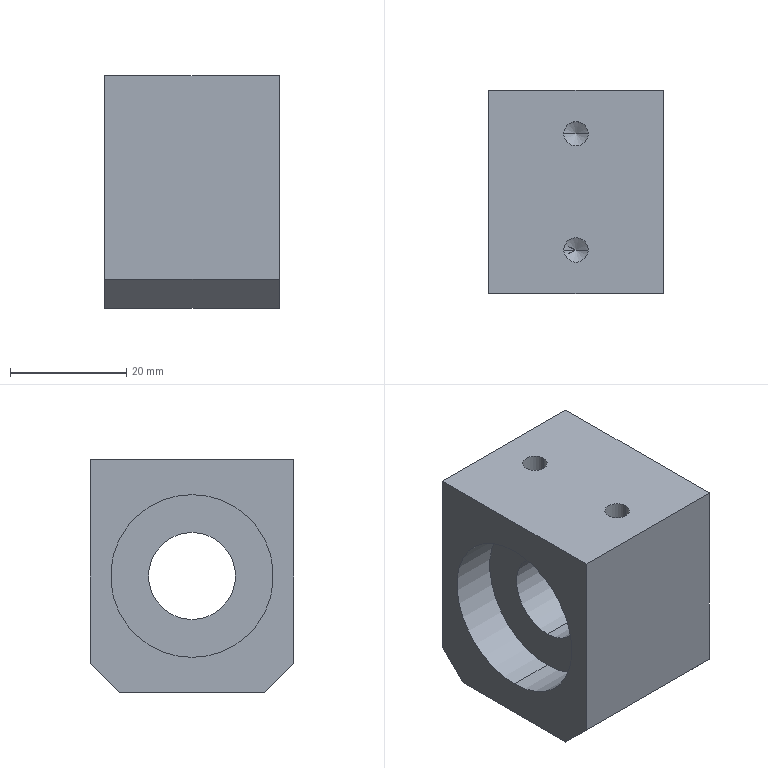Component | SolidWorks | ElectricalBoxAssembly2-1_AngleSensorComponentAssembly3-1_BearingHousing2-1 | 1 solid | 24 faces | box 30 x 35 x 40 mm | volume 28569 mm3 | cylinder 10 | plane 10 | cone 4 | commonest cylinder face diameters 4.2 x4 28 x4 15 x2
build123d program:
from build123d import *

# Parameters (mm, degrees)
SKETCH1_W             = 40
SKETCH1_H             = 35
BOSS_EXTRUDE1_DEPTH   = 15
SKETCH2_R             = 14
CUT_EXTRUDE1_DEPTH    = 8
SKETCH3_R             = 7.5
CUT_EXTRUDE2_DEPTH    = 35.5
M5_TAPPED_HOLE1_D     = 4.2
M5_TAPPED_HOLE1_DEPTH = 12.4
M5_TAPPED_HOLE1_TIP   = 1.262
CHAMFER1_SIZE         = 5


with BuildPart() as part:
    # Sketch1 → Boss-Extrude1 (new, symmetric)
    with BuildSketch(Plane.XY):
        Rectangle(SKETCH1_W, SKETCH1_H)
    extrude(amount=BOSS_EXTRUDE1_DEPTH, both=True)

    # Sketch2 → Cut-Extrude1 (cut)
    with BuildSketch(Plane.XY.offset(15)):
        Circle(SKETCH2_R)
    cut_extrude1 = extrude(amount=-CUT_EXTRUDE1_DEPTH, mode=Mode.SUBTRACT)

    # Mirror1: Cut-Extrude1 across plane
    add(cut_extrude1.mirror(Plane.XY), mode=Mode.SUBTRACT)

    # Sketch3 → Cut-Extrude2 (cut, through all)
    with BuildSketch(Plane.XY.offset(7)):
        Circle(SKETCH3_R)
    extrude(amount=-CUT_EXTRUDE2_DEPTH, mode=Mode.SUBTRACT)

    # M5 Tapped Hole1
    with Locations(Plane(origin=(20, 0, 0), x_dir=(0, 0, -1), z_dir=(1, 0, 0))):
        with Locations((0, 10), (0, -10)):
            Hole(M5_TAPPED_HOLE1_D / 2, depth=M5_TAPPED_HOLE1_DEPTH)
            with Locations((0, 0, -(M5_TAPPED_HOLE1_DEPTH + M5_TAPPED_HOLE1_TIP / 2))):  # 118° drill point
                Cone(0, M5_TAPPED_HOLE1_D / 2, M5_TAPPED_HOLE1_TIP, mode=Mode.SUBTRACT)

    # Chamfer1
    chamfer1_edges = [part.edges().sort_by_distance(p)[0] for p in [
        (-20, -17.5, 0),
        (-20, 17.5, 0),
    ]]
    chamfer(chamfer1_edges, length=CHAMFER1_SIZE)


solid = part.part

# Placed as in the assembly
solid = solid.moved(Location((824.115, 214.666, 1746.399), (0, -90, 0)))
STEP:
#1=COLOUR_RGB('',0.7922,0.8196,0.9333);
#2=FILL_AREA_STYLE_COLOUR('',#1);
#3=FILL_AREA_STYLE('',(#2));
#4=SURFACE_STYLE_FILL_AREA(#3);
#5=SURFACE_SIDE_STYLE('',(#4));
#6=SURFACE_STYLE_USAGE(.BOTH.,#5);
#7=PRESENTATION_STYLE_ASSIGNMENT((#6));
#8=CARTESIAN_POINT('',(32.363,8.845,69.055));
#9=VERTEX_POINT('',#8);
#10=CARTESIAN_POINT('',(32.528,8.845,69.055));
#11=VERTEX_POINT('',#10);
#12=CARTESIAN_POINT('',(32.445,8.845,69.055));
#13=DIRECTION('',(0.,0.,1.));
#14=DIRECTION('',(1.,0.,0.));
#15=AXIS2_PLACEMENT_3D('',#12,#13,#14);
#16=CIRCLE('',#15,0.08268);
#17=EDGE_CURVE('',#9,#11,#16,.T.);
#18=ORIENTED_EDGE('',*,*,#17,.F.);
#19=CARTESIAN_POINT('',(32.363,8.845,69.543));
#20=VERTEX_POINT('',#19);
#21=CARTESIAN_POINT('',(32.363,8.845,69.543));
#22=DIRECTION('',(0.,0.,1.));
#23=VECTOR('',#22,39.37);
#24=LINE('',#21,#23);
#25=EDGE_CURVE('',#9,#20,#24,.T.);
#26=ORIENTED_EDGE('',*,*,#25,.T.);
#27=CARTESIAN_POINT('',(32.528,8.845,69.543));
#28=VERTEX_POINT('',#27);
#29=CARTESIAN_POINT('',(32.445,8.845,69.543));
#30=DIRECTION('',(0.,0.,1.));
#31=DIRECTION('',(1.,0.,0.));
#32=AXIS2_PLACEMENT_3D('',#29,#30,#31);
#33=CIRCLE('',#32,0.08268);
#34=EDGE_CURVE('',#20,#28,#33,.T.);
#35=ORIENTED_EDGE('',*,*,#34,.T.);
#36=CARTESIAN_POINT('',(32.528,8.845,69.543));
#37=DIRECTION('',(0.,0.,1.));
#38=VECTOR('',#37,39.37);
#39=LINE('',#36,#38);
#40=EDGE_CURVE('',#11,#28,#39,.T.);
#41=ORIENTED_EDGE('',*,*,#40,.F.);
#42=EDGE_LOOP('',(#18,#26,#35,#41));
#43=FACE_OUTER_BOUND('',#42,.T.);
#44=CARTESIAN_POINT('',(32.445,8.845,69.543));
#45=DIRECTION('',(0.,0.,1.));
#46=DIRECTION('',(1.,0.,0.));
#47=AXIS2_PLACEMENT_3D('',#44,#45,#46);
#48=CYLINDRICAL_SURFACE('',#47,0.08268);
#49=ADVANCED_FACE('',(#43),#48,.F.);
#50=CARTESIAN_POINT('',(32.445,8.845,69.005));
#51=VERTEX_POINT('',#50);
#52=CARTESIAN_POINT('',(32.528,8.845,69.055));
#53=DIRECTION('',(0.8572,0.,0.515));
#54=VECTOR('',#53,39.37);
#55=LINE('',#52,#54);
#56=EDGE_CURVE('',#51,#11,#55,.T.);
#57=ORIENTED_EDGE('',*,*,#56,.F.);
#58=CARTESIAN_POINT('',(32.363,8.845,69.055));
#59=DIRECTION('',(-0.8572,0.,0.515));
#60=VECTOR('',#59,39.37);
#61=LINE('',#58,#60);
#62=EDGE_CURVE('',#51,#9,#61,.T.);
#63=ORIENTED_EDGE('',*,*,#62,.T.);
#64=ORIENTED_EDGE('',*,*,#17,.T.);
#65=EDGE_LOOP('',(#57,#63,#64));
#66=FACE_OUTER_BOUND('',#65,.T.);
#67=CARTESIAN_POINT('',(32.445,8.845,69.055));
#68=DIRECTION('',(0.,0.,1.));
#69=DIRECTION('',(1.,0.,0.));
#70=AXIS2_PLACEMENT_3D('',#67,#68,#69);
#71=CONICAL_SURFACE('',#70,0.08268,1.03);
#72=ADVANCED_FACE('',(#66),#71,.F.);
#73=CARTESIAN_POINT('',(32.363,8.058,69.055));
#74=VERTEX_POINT('',#73);
#75=CARTESIAN_POINT('',(32.528,8.058,69.055));
#76=VERTEX_POINT('',#75);
#77=CARTESIAN_POINT('',(32.445,8.058,69.055));
#78=DIRECTION('',(0.,0.,1.));
#79=DIRECTION('',(1.,0.,0.));
#80=AXIS2_PLACEMENT_3D('',#77,#78,#79);
#81=CIRCLE('',#80,0.08268);
#82=EDGE_CURVE('',#74,#76,#81,.T.);
#83=ORIENTED_EDGE('',*,*,#82,.F.);
#84=CARTESIAN_POINT('',(32.363,8.058,69.543));
#85=VERTEX_POINT('',#84);
#86=CARTESIAN_POINT('',(32.363,8.058,69.543));
#87=DIRECTION('',(0.,0.,1.));
#88=VECTOR('',#87,39.37);
#89=LINE('',#86,#88);
#90=EDGE_CURVE('',#74,#85,#89,.T.);
#91=ORIENTED_EDGE('',*,*,#90,.T.);
#92=CARTESIAN_POINT('',(32.528,8.058,69.543));
#93=VERTEX_POINT('',#92);
#94=CARTESIAN_POINT('',(32.445,8.058,69.543));
#95=DIRECTION('',(0.,0.,1.));
#96=DIRECTION('',(1.,0.,0.));
#97=AXIS2_PLACEMENT_3D('',#94,#95,#96);
#98=CIRCLE('',#97,0.08268);
#99=EDGE_CURVE('',#85,#93,#98,.T.);
#100=ORIENTED_EDGE('',*,*,#99,.T.);
#101=CARTESIAN_POINT('',(32.528,8.058,69.543));
#102=DIRECTION('',(0.,0.,1.));
#103=VECTOR('',#102,39.37);
#104=LINE('',#101,#103);
#105=EDGE_CURVE('',#76,#93,#104,.T.);
#106=ORIENTED_EDGE('',*,*,#105,.F.);
#107=EDGE_LOOP('',(#83,#91,#100,#106));
#108=FACE_OUTER_BOUND('',#107,.T.);
#109=CARTESIAN_POINT('',(32.445,8.058,69.543));
#110=DIRECTION('',(0.,0.,1.));
#111=DIRECTION('',(1.,0.,0.));
#112=AXIS2_PLACEMENT_3D('',#109,#110,#111);
#113=CYLINDRICAL_SURFACE('',#112,0.08268);
#114=ADVANCED_FACE('',(#108),#113,.F.);
#115=CARTESIAN_POINT('',(32.445,8.058,69.005));
#116=VERTEX_POINT('',#115);
#117=CARTESIAN_POINT('',(32.528,8.058,69.055));
#118=DIRECTION('',(0.8572,0.,0.515));
#119=VECTOR('',#118,39.37);
#120=LINE('',#117,#119);
#121=EDGE_CURVE('',#116,#76,#120,.T.);
#122=ORIENTED_EDGE('',*,*,#121,.F.);
#123=CARTESIAN_POINT('',(32.363,8.058,69.055));
#124=DIRECTION('',(-0.8572,0.,0.515));
#125=VECTOR('',#124,39.37);
#126=LINE('',#123,#125);
#127=EDGE_CURVE('',#116,#74,#126,.T.);
#128=ORIENTED_EDGE('',*,*,#127,.T.);
#129=ORIENTED_EDGE('',*,*,#82,.T.);
#130=EDGE_LOOP('',(#122,#128,#129));
#131=FACE_OUTER_BOUND('',#130,.T.);
#132=CARTESIAN_POINT('',(32.445,8.058,69.055));
#133=DIRECTION('',(0.,0.,1.));
#134=DIRECTION('',(1.,0.,0.));
#135=AXIS2_PLACEMENT_3D('',#132,#133,#134);
#136=CONICAL_SURFACE('',#135,0.08268,1.03);
#137=ADVANCED_FACE('',(#131),#136,.F.);
#138=CARTESIAN_POINT('',(32.721,8.451,69.051));
#139=VERTEX_POINT('',#138);
#140=CARTESIAN_POINT('',(32.721,8.451,68.461));
#141=VERTEX_POINT('',#140);
#142=CARTESIAN_POINT('',(32.721,8.451,68.756));
#143=DIRECTION('',(1.,0.,-0.));
#144=DIRECTION('',(-0.,-0.,-1.));
#145=AXIS2_PLACEMENT_3D('',#142,#143,#144);
#146=CIRCLE('',#145,0.2953);
#147=EDGE_CURVE('',#139,#141,#146,.T.);
#148=ORIENTED_EDGE('',*,*,#147,.T.);
#149=CARTESIAN_POINT('',(32.17,8.451,68.461));
#150=VERTEX_POINT('',#149);
#151=CARTESIAN_POINT('',(33.036,8.451,68.461));
#152=DIRECTION('',(-1.,-0.,0.));
#153=VECTOR('',#152,39.37);
#154=LINE('',#151,#153);
#155=EDGE_CURVE('',#141,#150,#154,.T.);
#156=ORIENTED_EDGE('',*,*,#155,.T.);
#157=CARTESIAN_POINT('',(32.17,8.451,69.051));
#158=VERTEX_POINT('',#157);
#159=CARTESIAN_POINT('',(32.17,8.451,68.756));
#160=DIRECTION('',(-1.,-0.,0.));
#161=DIRECTION('',(0.,0.,1.));
#162=AXIS2_PLACEMENT_3D('',#159,#160,#161);
#163=CIRCLE('',#162,0.2953);
#164=EDGE_CURVE('',#150,#158,#163,.T.);
#165=ORIENTED_EDGE('',*,*,#164,.T.);
#166=CARTESIAN_POINT('',(33.036,8.451,69.051));
#167=DIRECTION('',(-1.,-0.,0.));
#168=VECTOR('',#167,39.37);
#169=LINE('',#166,#168);
#170=EDGE_CURVE('',#139,#158,#169,.T.);
#171=ORIENTED_EDGE('',*,*,#170,.F.);
#172=EDGE_LOOP('',(#148,#156,#165,#171));
#173=FACE_OUTER_BOUND('',#172,.T.);
#174=CARTESIAN_POINT('',(33.036,8.451,68.756));
#175=DIRECTION('',(-1.,-0.,0.));
#176=DIRECTION('',(0.,0.,1.));
#177=AXIS2_PLACEMENT_3D('',#174,#175,#176);
#178=CYLINDRICAL_SURFACE('',#177,0.2953);
#179=ADVANCED_FACE('',(#173),#178,.F.);
#180=CARTESIAN_POINT('',(32.721,8.451,68.205));
#181=VERTEX_POINT('',#180);
#182=CARTESIAN_POINT('',(32.721,8.451,69.307));
#183=VERTEX_POINT('',#182);
#184=CARTESIAN_POINT('',(32.721,8.451,68.756));
#185=DIRECTION('',(-1.,-0.,0.));
#186=DIRECTION('',(0.,0.,1.));
#187=AXIS2_PLACEMENT_3D('',#184,#185,#186);
#188=CIRCLE('',#187,0.5512);
#189=EDGE_CURVE('',#181,#183,#188,.T.);
#190=ORIENTED_EDGE('',*,*,#189,.T.);
#191=CARTESIAN_POINT('',(33.036,8.451,69.307));
#192=VERTEX_POINT('',#191);
#193=CARTESIAN_POINT('',(32.721,8.451,69.307));
#194=DIRECTION('',(1.,0.,-0.));
#195=VECTOR('',#194,39.37);
#196=LINE('',#193,#195);
#197=EDGE_CURVE('',#183,#192,#196,.T.);
#198=ORIENTED_EDGE('',*,*,#197,.T.);
#199=CARTESIAN_POINT('',(33.036,8.451,68.205));
#200=VERTEX_POINT('',#199);
#201=CARTESIAN_POINT('',(33.036,8.451,68.756));
#202=DIRECTION('',(-1.,-0.,0.));
#203=DIRECTION('',(0.,0.,1.));
#204=AXIS2_PLACEMENT_3D('',#201,#202,#203);
#205=CIRCLE('',#204,0.5512);
#206=EDGE_CURVE('',#200,#192,#205,.T.);
#207=ORIENTED_EDGE('',*,*,#206,.F.);
#208=CARTESIAN_POINT('',(32.721,8.451,68.205));
#209=DIRECTION('',(1.,0.,-0.));
#210=VECTOR('',#209,39.37);
#211=LINE('',#208,#210);
#212=EDGE_CURVE('',#181,#200,#211,.T.);
#213=ORIENTED_EDGE('',*,*,#212,.F.);
#214=EDGE_LOOP('',(#190,#198,#207,#213));
#215=FACE_OUTER_BOUND('',#214,.T.);
#216=CARTESIAN_POINT('',(32.721,8.451,68.756));
#217=DIRECTION('',(1.,0.,-0.));
#218=DIRECTION('',(-0.,-0.,-1.));
#219=AXIS2_PLACEMENT_3D('',#216,#217,#218);
#220=CYLINDRICAL_SURFACE('',#219,0.5512);
#221=ADVANCED_FACE('',(#215),#220,.F.);
#222=CARTESIAN_POINT('',(32.17,8.451,68.205));
#223=VERTEX_POINT('',#222);
#224=CARTESIAN_POINT('',(32.17,8.451,69.307));
#225=VERTEX_POINT('',#224);
#226=CARTESIAN_POINT('',(32.17,8.451,68.756));
#227=DIRECTION('',(-1.,-0.,0.));
#228=DIRECTION('',(0.,0.,1.));
#229=AXIS2_PLACEMENT_3D('',#226,#227,#228);
#230=CIRCLE('',#229,0.5512);
#231=EDGE_CURVE('',#223,#225,#230,.T.);
#232=ORIENTED_EDGE('',*,*,#231,.F.);
#233=CARTESIAN_POINT('',(31.855,8.451,68.205));
#234=VERTEX_POINT('',#233);
#235=CARTESIAN_POINT('',(32.17,8.451,68.205));
#236=DIRECTION('',(-1.,-0.,0.));
#237=VECTOR('',#236,39.37);
#238=LINE('',#235,#237);
#239=EDGE_CURVE('',#223,#234,#238,.T.);
#240=ORIENTED_EDGE('',*,*,#239,.T.);
#241=CARTESIAN_POINT('',(31.855,8.451,69.307));
#242=VERTEX_POINT('',#241);
#243=CARTESIAN_POINT('',(31.855,8.451,68.756));
#244=DIRECTION('',(-1.,-0.,0.));
#245=DIRECTION('',(0.,0.,1.));
#246=AXIS2_PLACEMENT_3D('',#243,#244,#245);
#247=CIRCLE('',#246,0.5512);
#248=EDGE_CURVE('',#234,#242,#247,.T.);
#249=ORIENTED_EDGE('',*,*,#248,.T.);
#250=CARTESIAN_POINT('',(32.17,8.451,69.307));
#251=DIRECTION('',(-1.,-0.,0.));
#252=VECTOR('',#251,39.37);
#253=LINE('',#250,#252);
#254=EDGE_CURVE('',#225,#242,#253,.T.);
#255=ORIENTED_EDGE('',*,*,#254,.F.);
#256=EDGE_LOOP('',(#232,#240,#249,#255));
#257=FACE_OUTER_BOUND('',#256,.T.);
#258=CARTESIAN_POINT('',(32.17,8.451,68.756));
#259=DIRECTION('',(-1.,-0.,0.));
#260=DIRECTION('',(0.,0.,1.));
#261=AXIS2_PLACEMENT_3D('',#258,#259,#260);
#262=CYLINDRICAL_SURFACE('',#261,0.5512);
#263=ADVANCED_FACE('',(#257),#262,.F.);
#264=CARTESIAN_POINT('',(32.445,8.845,69.543));
#265=DIRECTION('',(0.,0.,1.));
#266=DIRECTION('',(1.,0.,0.));
#267=AXIS2_PLACEMENT_3D('',#264,#265,#266);
#268=CIRCLE('',#267,0.08268);
#269=EDGE_CURVE('',#28,#20,#268,.T.);
#270=ORIENTED_EDGE('',*,*,#269,.F.);
#271=ORIENTED_EDGE('',*,*,#34,.F.);
#272=EDGE_LOOP('',(#270,#271));
#273=FACE_BOUND('',#272,.T.);
#274=CARTESIAN_POINT('',(32.445,8.058,69.543));
#275=DIRECTION('',(0.,0.,1.));
#276=DIRECTION('',(1.,0.,0.));
#277=AXIS2_PLACEMENT_3D('',#274,#275,#276);
#278=CIRCLE('',#277,0.08268);
#279=EDGE_CURVE('',#93,#85,#278,.T.);
#280=ORIENTED_EDGE('',*,*,#279,.F.);
#281=ORIENTED_EDGE('',*,*,#99,.F.);
#282=EDGE_LOOP('',(#280,#281));
#283=FACE_BOUND('',#282,.T.);
#284=CARTESIAN_POINT('',(33.036,7.762,69.543));
#285=VERTEX_POINT('',#284);
#286=CARTESIAN_POINT('',(33.036,9.14,69.543));
#287=VERTEX_POINT('',#286);
#288=CARTESIAN_POINT('',(33.036,9.14,69.543));
#289=DIRECTION('',(-0.,1.,-0.));
#290=VECTOR('',#289,39.37);
#291=LINE('',#288,#290);
#292=EDGE_CURVE('',#285,#287,#291,.T.);
#293=ORIENTED_EDGE('',*,*,#292,.T.);
#294=CARTESIAN_POINT('',(31.855,9.14,69.543));
#295=VERTEX_POINT('',#294);
#296=CARTESIAN_POINT('',(31.855,9.14,69.543));
#297=DIRECTION('',(1.,0.,-0.));
#298=VECTOR('',#297,39.37);
#299=LINE('',#296,#298);
#300=EDGE_CURVE('',#295,#287,#299,.T.);
#301=ORIENTED_EDGE('',*,*,#300,.F.);
#302=CARTESIAN_POINT('',(31.855,7.762,69.543));
#303=VERTEX_POINT('',#302);
#304=CARTESIAN_POINT('',(31.855,9.14,69.543));
#305=DIRECTION('',(-0.,1.,-0.));
#306=VECTOR('',#305,39.37);
#307=LINE('',#304,#306);
#308=EDGE_CURVE('',#303,#295,#307,.T.);
#309=ORIENTED_EDGE('',*,*,#308,.F.);
#310=CARTESIAN_POINT('',(31.855,7.762,69.543));
#311=DIRECTION('',(1.,0.,-0.));
#312=VECTOR('',#311,39.37);
#313=LINE('',#310,#312);
#314=EDGE_CURVE('',#303,#285,#313,.T.);
#315=ORIENTED_EDGE('',*,*,#314,.T.);
#316=EDGE_LOOP('',(#293,#301,#309,#315));
#317=FACE_OUTER_BOUND('',#316,.T.);
#318=CARTESIAN_POINT('',(31.855,9.14,69.543));
#319=DIRECTION('',(-0.,-0.,-1.));
#320=DIRECTION('',(0.,-1.,0.));
#321=AXIS2_PLACEMENT_3D('',#318,#319,#320);
#322=PLANE('',#321);
#323=ADVANCED_FACE('',(#273,#283,#317),#322,.F.);
#324=CARTESIAN_POINT('',(33.036,9.14,68.165));
#325=VERTEX_POINT('',#324);
#326=CARTESIAN_POINT('',(33.036,9.14,67.968));
#327=DIRECTION('',(-0.,-0.,-1.));
#328=VECTOR('',#327,39.37);
#329=LINE('',#326,#328);
#330=EDGE_CURVE('',#287,#325,#329,.T.);
#331=ORIENTED_EDGE('',*,*,#330,.T.);
#332=CARTESIAN_POINT('',(31.855,9.14,68.165));
#333=VERTEX_POINT('',#332);
#334=CARTESIAN_POINT('',(31.855,9.14,68.165));
#335=DIRECTION('',(-1.,-0.,0.));
#336=VECTOR('',#335,39.37);
#337=LINE('',#334,#336);
#338=EDGE_CURVE('',#325,#333,#337,.T.);
#339=ORIENTED_EDGE('',*,*,#338,.T.);
#340=CARTESIAN_POINT('',(31.855,9.14,67.968));
#341=DIRECTION('',(-0.,-0.,-1.));
#342=VECTOR('',#341,39.37);
#343=LINE('',#340,#342);
#344=EDGE_CURVE('',#295,#333,#343,.T.);
#345=ORIENTED_EDGE('',*,*,#344,.F.);
#346=ORIENTED_EDGE('',*,*,#300,.T.);
#347=EDGE_LOOP('',(#331,#339,#345,#346));
#348=FACE_OUTER_BOUND('',#347,.T.);
#349=CARTESIAN_POINT('',(31.855,9.14,67.968));
#350=DIRECTION('',(0.,-1.,0.));
#351=DIRECTION('',(1.,0.,-0.));
#352=AXIS2_PLACEMENT_3D('',#349,#350,#351);
#353=PLANE('',#352);
#354=ADVANCED_FACE('',(#348),#353,.F.);
#355=CARTESIAN_POINT('',(31.855,8.944,67.968));
#356=VERTEX_POINT('',#355);
#357=CARTESIAN_POINT('',(31.855,7.959,67.968));
#358=VERTEX_POINT('',#357);
#359=CARTESIAN_POINT('',(31.855,9.14,67.968));
#360=DIRECTION('',(0.,-1.,0.));
#361=VECTOR('',#360,39.37);
#362=LINE('',#359,#361);
#363=EDGE_CURVE('',#356,#358,#362,.T.);
#364=ORIENTED_EDGE('',*,*,#363,.F.);
#365=CARTESIAN_POINT('',(33.036,8.944,67.968));
#366=VERTEX_POINT('',#365);
#367=CARTESIAN_POINT('',(31.855,8.944,67.968));
#368=DIRECTION('',(1.,0.,-0.));
#369=VECTOR('',#368,39.37);
#370=LINE('',#367,#369);
#371=EDGE_CURVE('',#356,#366,#370,.T.);
#372=ORIENTED_EDGE('',*,*,#371,.T.);
#373=CARTESIAN_POINT('',(33.036,7.959,67.968));
#374=VERTEX_POINT('',#373);
#375=CARTESIAN_POINT('',(33.036,9.14,67.968));
#376=DIRECTION('',(0.,-1.,0.));
#377=VECTOR('',#376,39.37);
#378=LINE('',#375,#377);
#379=EDGE_CURVE('',#366,#374,#378,.T.);
#380=ORIENTED_EDGE('',*,*,#379,.T.);
#381=CARTESIAN_POINT('',(31.855,7.959,67.968));
#382=DIRECTION('',(-1.,-0.,0.));
#383=VECTOR('',#382,39.37);
#384=LINE('',#381,#383);
#385=EDGE_CURVE('',#374,#358,#384,.T.);
#386=ORIENTED_EDGE('',*,*,#385,.T.);
#387=EDGE_LOOP('',(#364,#372,#380,#386));
#388=FACE_OUTER_BOUND('',#387,.T.);
#389=CARTESIAN_POINT('',(31.855,9.14,67.968));
#390=DIRECTION('',(0.,0.,1.));
#391=DIRECTION('',(-0.,1.,-0.));
#392=AXIS2_PLACEMENT_3D('',#389,#390,#391);
#393=PLANE('',#392);
#394=ADVANCED_FACE('',(#388),#393,.F.);
#395=CARTESIAN_POINT('',(31.855,7.762,68.165));
#396=VERTEX_POINT('',#395);
#397=CARTESIAN_POINT('',(31.855,7.762,67.968));
#398=DIRECTION('',(0.,0.,1.));
#399=VECTOR('',#398,39.37);
#400=LINE('',#397,#399);
#401=EDGE_CURVE('',#396,#303,#400,.T.);
#402=ORIENTED_EDGE('',*,*,#401,.F.);
#403=CARTESIAN_POINT('',(33.036,7.762,68.165));
#404=VERTEX_POINT('',#403);
#405=CARTESIAN_POINT('',(31.855,7.762,68.165));
#406=DIRECTION('',(1.,0.,-0.));
#407=VECTOR('',#406,39.37);
#408=LINE('',#405,#407);
#409=EDGE_CURVE('',#396,#404,#408,.T.);
#410=ORIENTED_EDGE('',*,*,#409,.T.);
#411=CARTESIAN_POINT('',(33.036,7.762,67.968));
#412=DIRECTION('',(0.,0.,1.));
#413=VECTOR('',#412,39.37);
#414=LINE('',#411,#413);
#415=EDGE_CURVE('',#404,#285,#414,.T.);
#416=ORIENTED_EDGE('',*,*,#415,.T.);
#417=ORIENTED_EDGE('',*,*,#314,.F.);
#418=EDGE_LOOP('',(#402,#410,#416,#417));
#419=FACE_OUTER_BOUND('',#418,.T.);
#420=CARTESIAN_POINT('',(31.855,7.762,67.968));
#421=DIRECTION('',(-0.,1.,-0.));
#422=DIRECTION('',(-1.,-0.,0.));
#423=AXIS2_PLACEMENT_3D('',#420,#421,#422);
#424=PLANE('',#423);
#425=ADVANCED_FACE('',(#419),#424,.F.);
#426=CARTESIAN_POINT('',(31.855,8.451,68.756));
#427=DIRECTION('',(-1.,-0.,0.));
#428=DIRECTION('',(0.,0.,1.));
#429=AXIS2_PLACEMENT_3D('',#426,#427,#428);
#430=CIRCLE('',#429,0.5512);
#431=EDGE_CURVE('',#242,#234,#430,.T.);
#432=ORIENTED_EDGE('',*,*,#431,.F.);
#433=ORIENTED_EDGE('',*,*,#248,.F.);
#434=EDGE_LOOP('',(#432,#433));
#435=FACE_BOUND('',#434,.T.);
#436=ORIENTED_EDGE('',*,*,#344,.T.);
#437=CARTESIAN_POINT('',(31.855,9.091,68.116));
#438=DIRECTION('',(-0.,-0.7071,-0.7071));
#439=VECTOR('',#438,39.37);
#440=LINE('',#437,#439);
#441=EDGE_CURVE('',#333,#356,#440,.T.);
#442=ORIENTED_EDGE('',*,*,#441,.T.);
#443=ORIENTED_EDGE('',*,*,#363,.T.);
#444=CARTESIAN_POINT('',(31.855,7.812,68.116));
#445=DIRECTION('',(0.,-0.7071,0.7071));
#446=VECTOR('',#445,39.37);
#447=LINE('',#444,#446);
#448=EDGE_CURVE('',#358,#396,#447,.T.);
#449=ORIENTED_EDGE('',*,*,#448,.T.);
#450=ORIENTED_EDGE('',*,*,#401,.T.);
#451=ORIENTED_EDGE('',*,*,#308,.T.);
#452=EDGE_LOOP('',(#436,#442,#443,#449,#450,#451));
#453=FACE_OUTER_BOUND('',#452,.T.);
#454=CARTESIAN_POINT('',(31.855,8.451,68.756));
#455=DIRECTION('',(-1.,-0.,0.));
#456=DIRECTION('',(0.,0.,1.));
#457=AXIS2_PLACEMENT_3D('',#454,#455,#456);
#458=PLANE('',#457);
#459=ADVANCED_FACE('',(#435,#453),#458,.T.);
#460=ORIENTED_EDGE('',*,*,#206,.T.);
#461=CARTESIAN_POINT('',(33.036,8.451,68.756));
#462=DIRECTION('',(-1.,-0.,0.));
#463=DIRECTION('',(0.,0.,1.));
#464=AXIS2_PLACEMENT_3D('',#461,#462,#463);
#465=CIRCLE('',#464,0.5512);
#466=EDGE_CURVE('',#192,#200,#465,.T.);
#467=ORIENTED_EDGE('',*,*,#466,.T.);
#468=EDGE_LOOP('',(#460,#467));
#469=FACE_BOUND('',#468,.T.);
#470=ORIENTED_EDGE('',*,*,#379,.F.);
#471=CARTESIAN_POINT('',(33.036,8.944,67.968));
#472=DIRECTION('',(0.,0.7071,0.7071));
#473=VECTOR('',#472,39.37);
#474=LINE('',#471,#473);
#475=EDGE_CURVE('',#366,#325,#474,.T.);
#476=ORIENTED_EDGE('',*,*,#475,.T.);
#477=ORIENTED_EDGE('',*,*,#330,.F.);
#478=ORIENTED_EDGE('',*,*,#292,.F.);
#479=ORIENTED_EDGE('',*,*,#415,.F.);
#480=CARTESIAN_POINT('',(33.036,7.762,68.165));
#481=DIRECTION('',(-0.,0.7071,-0.7071));
#482=VECTOR('',#481,39.37);
#483=LINE('',#480,#482);
#484=EDGE_CURVE('',#404,#374,#483,.T.);
#485=ORIENTED_EDGE('',*,*,#484,.T.);
#486=EDGE_LOOP('',(#470,#476,#477,#478,#479,#485));
#487=FACE_OUTER_BOUND('',#486,.T.);
#488=CARTESIAN_POINT('',(33.036,8.451,68.756));
#489=DIRECTION('',(-1.,-0.,0.));
#490=DIRECTION('',(0.,0.,1.));
#491=AXIS2_PLACEMENT_3D('',#488,#489,#490);
#492=PLANE('',#491);
#493=ADVANCED_FACE('',(#469,#487),#492,.F.);
#494=ORIENTED_EDGE('',*,*,#239,.F.);
#495=CARTESIAN_POINT('',(32.17,8.451,68.756));
#496=DIRECTION('',(-1.,-0.,0.));
#497=DIRECTION('',(0.,0.,1.));
#498=AXIS2_PLACEMENT_3D('',#495,#496,#497);
#499=CIRCLE('',#498,0.5512);
#500=EDGE_CURVE('',#225,#223,#499,.T.);
#501=ORIENTED_EDGE('',*,*,#500,.F.);
#502=ORIENTED_EDGE('',*,*,#254,.T.);
#503=ORIENTED_EDGE('',*,*,#431,.T.);
#504=EDGE_LOOP('',(#494,#501,#502,#503));
#505=FACE_OUTER_BOUND('',#504,.T.);
#506=CARTESIAN_POINT('',(32.17,8.451,68.756));
#507=DIRECTION('',(-1.,-0.,0.));
#508=DIRECTION('',(0.,0.,1.));
#509=AXIS2_PLACEMENT_3D('',#506,#507,#508);
#510=CYLINDRICAL_SURFACE('',#509,0.5512);
#511=ADVANCED_FACE('',(#505),#510,.F.);
#512=CARTESIAN_POINT('',(32.17,8.451,68.756));
#513=DIRECTION('',(-1.,-0.,0.));
#514=DIRECTION('',(0.,0.,1.));
#515=AXIS2_PLACEMENT_3D('',#512,#513,#514);
#516=CIRCLE('',#515,0.2953);
#517=EDGE_CURVE('',#158,#150,#516,.T.);
#518=ORIENTED_EDGE('',*,*,#517,.F.);
#519=ORIENTED_EDGE('',*,*,#164,.F.);
#520=EDGE_LOOP('',(#518,#519));
#521=FACE_BOUND('',#520,.T.);
#522=ORIENTED_EDGE('',*,*,#500,.T.);
#523=ORIENTED_EDGE('',*,*,#231,.T.);
#524=EDGE_LOOP('',(#522,#523));
#525=FACE_OUTER_BOUND('',#524,.T.);
#526=CARTESIAN_POINT('',(32.17,8.451,68.756));
#527=DIRECTION('',(-1.,-0.,0.));
#528=DIRECTION('',(0.,0.,1.));
#529=AXIS2_PLACEMENT_3D('',#526,#527,#528);
#530=PLANE('',#529);
#531=ADVANCED_FACE('',(#521,#525),#530,.T.);
#532=ORIENTED_EDGE('',*,*,#197,.F.);
#533=CARTESIAN_POINT('',(32.721,8.451,68.756));
#534=DIRECTION('',(-1.,-0.,0.));
#535=DIRECTION('',(0.,0.,1.));
#536=AXIS2_PLACEMENT_3D('',#533,#534,#535);
#537=CIRCLE('',#536,0.5512);
#538=EDGE_CURVE('',#183,#181,#537,.T.);
#539=ORIENTED_EDGE('',*,*,#538,.T.);
#540=ORIENTED_EDGE('',*,*,#212,.T.);
#541=ORIENTED_EDGE('',*,*,#466,.F.);
#542=EDGE_LOOP('',(#532,#539,#540,#541));
#543=FACE_OUTER_BOUND('',#542,.T.);
#544=CARTESIAN_POINT('',(32.721,8.451,68.756));
#545=DIRECTION('',(1.,0.,-0.));
#546=DIRECTION('',(-0.,-0.,-1.));
#547=AXIS2_PLACEMENT_3D('',#544,#545,#546);
#548=CYLINDRICAL_SURFACE('',#547,0.5512);
#549=ADVANCED_FACE('',(#543),#548,.F.);
#550=ORIENTED_EDGE('',*,*,#147,.F.);
#551=CARTESIAN_POINT('',(32.721,8.451,68.756));
#552=DIRECTION('',(1.,0.,-0.));
#553=DIRECTION('',(-0.,-0.,-1.));
#554=AXIS2_PLACEMENT_3D('',#551,#552,#553);
#555=CIRCLE('',#554,0.2953);
#556=EDGE_CURVE('',#141,#139,#555,.T.);
#557=ORIENTED_EDGE('',*,*,#556,.F.);
#558=EDGE_LOOP('',(#550,#557));
#559=FACE_BOUND('',#558,.T.);
#560=ORIENTED_EDGE('',*,*,#189,.F.);
#561=ORIENTED_EDGE('',*,*,#538,.F.);
#562=EDGE_LOOP('',(#560,#561));
#563=FACE_OUTER_BOUND('',#562,.T.);
#564=CARTESIAN_POINT('',(32.721,8.451,68.756));
#565=DIRECTION('',(1.,0.,-0.));
#566=DIRECTION('',(0.,0.,1.));
#567=AXIS2_PLACEMENT_3D('',#564,#565,#566);
#568=PLANE('',#567);
#569=ADVANCED_FACE('',(#559,#563),#568,.T.);
#570=ORIENTED_EDGE('',*,*,#155,.F.);
#571=ORIENTED_EDGE('',*,*,#556,.T.);
#572=ORIENTED_EDGE('',*,*,#170,.T.);
#573=ORIENTED_EDGE('',*,*,#517,.T.);
#574=EDGE_LOOP('',(#570,#571,#572,#573));
#575=FACE_OUTER_BOUND('',#574,.T.);
#576=CARTESIAN_POINT('',(33.036,8.451,68.756));
#577=DIRECTION('',(-1.,-0.,0.));
#578=DIRECTION('',(0.,0.,1.));
#579=AXIS2_PLACEMENT_3D('',#576,#577,#578);
#580=CYLINDRICAL_SURFACE('',#579,0.2953);
#581=ADVANCED_FACE('',(#575),#580,.F.);
#582=ORIENTED_EDGE('',*,*,#127,.F.);
#583=ORIENTED_EDGE('',*,*,#121,.T.);
#584=CARTESIAN_POINT('',(32.445,8.058,69.055));
#585=DIRECTION('',(0.,0.,1.));
#586=DIRECTION('',(1.,0.,0.));
#587=AXIS2_PLACEMENT_3D('',#584,#585,#586);
#588=CIRCLE('',#587,0.08268);
#589=EDGE_CURVE('',#76,#74,#588,.T.);
#590=ORIENTED_EDGE('',*,*,#589,.T.);
#591=EDGE_LOOP('',(#582,#583,#590));
#592=FACE_OUTER_BOUND('',#591,.T.);
#593=CARTESIAN_POINT('',(32.445,8.058,69.055));
#594=DIRECTION('',(0.,0.,1.));
#595=DIRECTION('',(1.,0.,0.));
#596=AXIS2_PLACEMENT_3D('',#593,#594,#595);
#597=CONICAL_SURFACE('',#596,0.08268,1.03);
#598=ADVANCED_FACE('',(#592),#597,.F.);
#599=ORIENTED_EDGE('',*,*,#90,.F.);
#600=ORIENTED_EDGE('',*,*,#589,.F.);
#601=ORIENTED_EDGE('',*,*,#105,.T.);
#602=ORIENTED_EDGE('',*,*,#279,.T.);
#603=EDGE_LOOP('',(#599,#600,#601,#602));
#604=FACE_OUTER_BOUND('',#603,.T.);
#605=CARTESIAN_POINT('',(32.445,8.058,69.543));
#606=DIRECTION('',(0.,0.,1.));
#607=DIRECTION('',(1.,0.,0.));
#608=AXIS2_PLACEMENT_3D('',#605,#606,#607);
#609=CYLINDRICAL_SURFACE('',#608,0.08268);
#610=ADVANCED_FACE('',(#604),#609,.F.);
#611=ORIENTED_EDGE('',*,*,#62,.F.);
#612=ORIENTED_EDGE('',*,*,#56,.T.);
#613=CARTESIAN_POINT('',(32.445,8.845,69.055));
#614=DIRECTION('',(0.,0.,1.));
#615=DIRECTION('',(1.,0.,0.));
#616=AXIS2_PLACEMENT_3D('',#613,#614,#615);
#617=CIRCLE('',#616,0.08268);
#618=EDGE_CURVE('',#11,#9,#617,.T.);
#619=ORIENTED_EDGE('',*,*,#618,.T.);
#620=EDGE_LOOP('',(#611,#612,#619));
#621=FACE_OUTER_BOUND('',#620,.T.);
#622=CARTESIAN_POINT('',(32.445,8.845,69.055));
#623=DIRECTION('',(0.,0.,1.));
#624=DIRECTION('',(1.,0.,0.));
#625=AXIS2_PLACEMENT_3D('',#622,#623,#624);
#626=CONICAL_SURFACE('',#625,0.08268,1.03);
#627=ADVANCED_FACE('',(#621),#626,.F.);
#628=ORIENTED_EDGE('',*,*,#25,.F.);
#629=ORIENTED_EDGE('',*,*,#618,.F.);
#630=ORIENTED_EDGE('',*,*,#40,.T.);
#631=ORIENTED_EDGE('',*,*,#269,.T.);
#632=EDGE_LOOP('',(#628,#629,#630,#631));
#633=FACE_OUTER_BOUND('',#632,.T.);
#634=CARTESIAN_POINT('',(32.445,8.845,69.543));
#635=DIRECTION('',(0.,0.,1.));
#636=DIRECTION('',(1.,0.,0.));
#637=AXIS2_PLACEMENT_3D('',#634,#635,#636);
#638=CYLINDRICAL_SURFACE('',#637,0.08268);
#639=ADVANCED_FACE('',(#633),#638,.F.);
#640=ORIENTED_EDGE('',*,*,#441,.F.);
#641=ORIENTED_EDGE('',*,*,#338,.F.);
#642=ORIENTED_EDGE('',*,*,#475,.F.);
#643=ORIENTED_EDGE('',*,*,#371,.F.);
#644=EDGE_LOOP('',(#640,#641,#642,#643));
#645=FACE_OUTER_BOUND('',#644,.T.);
#646=CARTESIAN_POINT('',(31.855,8.944,67.968));
#647=DIRECTION('',(0.,-0.7071,0.7071));
#648=DIRECTION('',(1.,0.,-0.));
#649=AXIS2_PLACEMENT_3D('',#646,#647,#648);
#650=PLANE('',#649);
#651=ADVANCED_FACE('',(#645),#650,.F.);
#652=ORIENTED_EDGE('',*,*,#448,.F.);
#653=ORIENTED_EDGE('',*,*,#385,.F.);
#654=ORIENTED_EDGE('',*,*,#484,.F.);
#655=ORIENTED_EDGE('',*,*,#409,.F.);
#656=EDGE_LOOP('',(#652,#653,#654,#655));
#657=FACE_OUTER_BOUND('',#656,.T.);
#658=CARTESIAN_POINT('',(31.855,7.762,68.165));
#659=DIRECTION('',(0.,0.7071,0.7071));
#660=DIRECTION('',(1.,0.,-0.));
#661=AXIS2_PLACEMENT_3D('',#658,#659,#660);
#662=PLANE('',#661);
#663=ADVANCED_FACE('',(#657),#662,.F.);
#664=CLOSED_SHELL('',(#49,#72,#114,#137,#179,#221,#263,#323,#354,#394,#425,#459,#493,#511,#531,#549,#569,#581,#598,#610,#627,#639,#651,#663));
#665=MANIFOLD_SOLID_BREP('',#664);
#666=STYLED_ITEM('',(#7),#665);
#667=PRESENTATION_LAYER_ASSIGNMENT('','',(#666));
#668=CARTESIAN_POINT('',(0.,0.,0.));
#669=DIRECTION('',(0.,0.,1.));
#670=DIRECTION('',(1.,0.,0.));
#671=AXIS2_PLACEMENT_3D('',#668,#669,#670);
#672=(LENGTH_UNIT()NAMED_UNIT(*)SI_UNIT($,.METRE.));
#673=LENGTH_MEASURE_WITH_UNIT(LENGTH_MEASURE(0.0254),#672);
#674=DIMENSIONAL_EXPONENTS(1.,0.,0.,0.,0.,0.,0.);
#675=(CONVERSION_BASED_UNIT('',#673)LENGTH_UNIT()NAMED_UNIT(#674));
#676=UNCERTAINTY_MEASURE_WITH_UNIT(LENGTH_MEASURE(0.00001),#675,'','');
#677=(NAMED_UNIT(*)PLANE_ANGLE_UNIT()SI_UNIT($,.RADIAN.));
#678=(NAMED_UNIT(*)SI_UNIT($,.STERADIAN.)SOLID_ANGLE_UNIT());
#679=(GEOMETRIC_REPRESENTATION_CONTEXT(3)GLOBAL_UNCERTAINTY_ASSIGNED_CONTEXT((#676))GLOBAL_UNIT_ASSIGNED_CONTEXT((#675,#677,#678))REPRESENTATION_CONTEXT('',''));
#680=ADVANCED_BREP_SHAPE_REPRESENTATION('',(#665,#671),#679);
#681=(LENGTH_UNIT()NAMED_UNIT(*)SI_UNIT($,.METRE.));
#682=LENGTH_MEASURE_WITH_UNIT(LENGTH_MEASURE(0.0254),#681);
#683=DIMENSIONAL_EXPONENTS(1.,0.,0.,0.,0.,0.,0.);
#684=(CONVERSION_BASED_UNIT('',#682)LENGTH_UNIT()NAMED_UNIT(#683));
#685=UNCERTAINTY_MEASURE_WITH_UNIT(LENGTH_MEASURE(0.00001),#684,'','');
#686=(NAMED_UNIT(*)PLANE_ANGLE_UNIT()SI_UNIT($,.RADIAN.));
#687=(NAMED_UNIT(*)SI_UNIT($,.STERADIAN.)SOLID_ANGLE_UNIT());
#688=(GEOMETRIC_REPRESENTATION_CONTEXT(3)GLOBAL_UNCERTAINTY_ASSIGNED_CONTEXT((#685))GLOBAL_UNIT_ASSIGNED_CONTEXT((#684,#686,#687))REPRESENTATION_CONTEXT('',''));
#689=MECHANICAL_DESIGN_GEOMETRIC_PRESENTATION_REPRESENTATION('',(#666),#688);